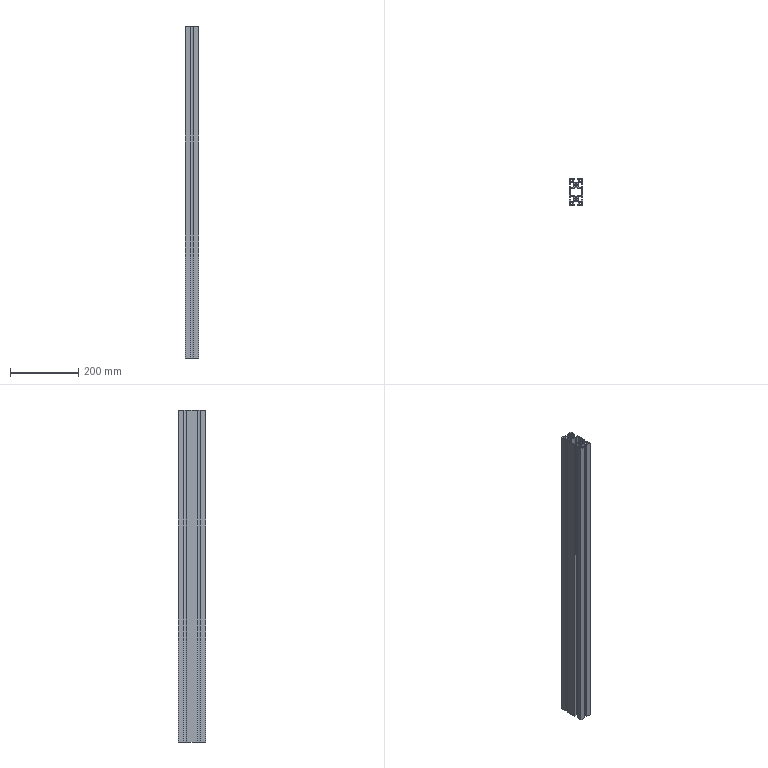Component | SolidWorks | 30-01A-1_EF4080-1080-1 | 1 solid | 84 faces | box 40 x 80 x 970 mm | volume 1116515 mm3 | plane 58 | cylinder 26 | commonest cylinder face diameters 8 x12 19 x10 6.8 x4
build123d program:
from build123d import *

# Parameters (mm, degrees)
SKETCH1_R      = 4
SKETCH1_R_2    = 3.4
EXTRUDE1_DEPTH = 485


with BuildPart() as part:
    # Sketch1 → Extrude1 (new, symmetric)
    with BuildSketch(Plane(origin=(0, 0, 0), x_dir=(0, 0, -1), z_dir=(0, 1, 0))):
        with BuildLine():
            Line((-40, 20), (-24.2, 20))
            Line((-24.2, 20), (-24.2, 16))
            Line((-24.2, 16), (-27.25, 16))
            Line((-27.25, 16), (-27.25, 9.361))
            ThreePointArc((-27.25, 9.361), (-20, 6), (-12.75, 9.361))
            Line((-12.75, 9.361), (-12.75, 16))
            Line((-12.75, 16), (-15.8, 16))
            Line((-15.8, 16), (-15.8, 20))
            Line((-15.8, 20), (15.8, 20))
            Line((15.8, 20), (15.8, 16))
            Line((15.8, 16), (12.75, 16))
            Line((12.75, 16), (12.75, 9.361))
            ThreePointArc((12.75, 9.361), (20, 6), (27.25, 9.361))
            Line((27.25, 9.361), (27.25, 16))
            Line((27.25, 16), (24.2, 16))
            Line((24.2, 16), (24.2, 20))
            Line((24.2, 20), (40, 20))
            Line((40, 20), (40, 4.2))
            Line((40, 4.2), (36, 4.2))
            Line((36, 4.2), (36, 7.25))
            Line((36, 7.25), (29.361, 7.25))
            ThreePointArc((29.361, 7.25), (26, 0), (29.361, -7.25))
            Line((29.361, -7.25), (36, -7.25))
            Line((36, -7.25), (36, -4.2))
            Line((36, -4.2), (40, -4.2))
            Line((40, -4.2), (40, -20))
            Line((40, -20), (24.2, -20))
            Line((24.2, -20), (24.2, -16))
            Line((24.2, -16), (27.25, -16))
            Line((27.25, -16), (27.25, -9.361))
            ThreePointArc((27.25, -9.361), (20, -6), (12.75, -9.361))
            Line((12.75, -9.361), (12.75, -16))
            Line((12.75, -16), (15.8, -16))
            Line((15.8, -16), (15.8, -20))
            Line((15.8, -20), (-15.8, -20))
            Line((-15.8, -20), (-15.8, -16))
            Line((-15.8, -16), (-12.75, -16))
            Line((-12.75, -16), (-12.75, -9.361))
            ThreePointArc((-12.75, -9.361), (-20, -6), (-27.25, -9.361))
            Line((-27.25, -9.361), (-27.25, -16))
            Line((-27.25, -16), (-24.2, -16))
            Line((-24.2, -16), (-24.2, -20))
            Line((-24.2, -20), (-40, -20))
            Line((-40, -20), (-40, -4.2))
            Line((-40, -4.2), (-36, -4.2))
            Line((-36, -4.2), (-36, -7.25))
            Line((-36, -7.25), (-29.361, -7.25))
            ThreePointArc((-29.361, -7.25), (-26, 0), (-29.361, 7.25))
            Line((-29.361, 7.25), (-36, 7.25))
            Line((-36, 7.25), (-36, 4.2))
            Line((-36, 4.2), (-40, 4.2))
            Line((-40, 4.2), (-40, 20))
        make_face()
        with Locations(Location((-33.5, 13.5, 0), (0, 0, 180))):
            Circle(SKETCH1_R, mode=Mode.SUBTRACT)
        with Locations(Location((-20, 0, 0), (0, 0, 180))):
            Circle(SKETCH1_R_2, mode=Mode.SUBTRACT)
        with Locations((-33.5, -13.5)):
            Circle(SKETCH1_R, mode=Mode.SUBTRACT)
        with Locations(Location((33.5, -13.5, 0), (0, 0, 180))):
            Circle(SKETCH1_R, mode=Mode.SUBTRACT)
        with Locations((20, 0)):
            Circle(SKETCH1_R_2, mode=Mode.SUBTRACT)
        with Locations((33.5, 13.5)):
            Circle(SKETCH1_R, mode=Mode.SUBTRACT)
        with BuildLine():
            Line((-10.5, -7.25), (-10.5, -13.5))
            ThreePointArc((-10.5, -13.5), (-9.328, -16.328), (-6.5, -17.5))
            Line((-6.5, -17.5), (6.5, -17.5))
            ThreePointArc((6.5, -17.5), (9.328, -16.328), (10.5, -13.5))
            Line((10.5, -13.5), (10.5, -7.25))
            Line((10.5, -7.25), (10.639, -7.25))
            ThreePointArc((10.639, -7.25), (14, 0), (10.639, 7.25))
            Line((10.639, 7.25), (10.5, 7.25))
            Line((10.5, 7.25), (10.5, 13.5))
            ThreePointArc((10.5, 13.5), (9.328, 16.328), (6.5, 17.5))
            Line((6.5, 17.5), (-6.5, 17.5))
            ThreePointArc((-6.5, 17.5), (-9.328, 16.328), (-10.5, 13.5))
            Line((-10.5, 13.5), (-10.5, 7.25))
            Line((-10.5, 7.25), (-10.639, 7.25))
            ThreePointArc((-10.639, 7.25), (-14, 0), (-10.639, -7.25))
            Line((-10.639, -7.25), (-10.5, -7.25))
        make_face(mode=Mode.SUBTRACT)
    extrude(amount=EXTRUDE1_DEPTH, both=True)


solid = part.part

# Placed as in the assembly
solid = solid.moved(Location((-427.43, 392.155, -525), (90, 0, 0)))